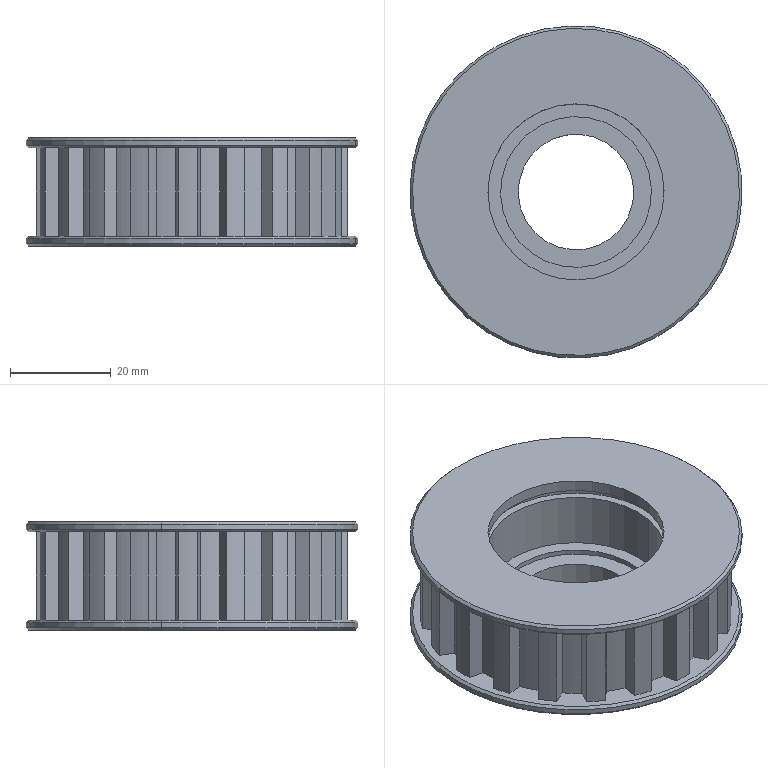Component | SolidWorks | DoubleFilmTransport-1_DrivenWheel-1 | 1 solid | 111 faces | volume 43508 mm3 | cylinder 55 | plane 48 | cone 8 | commonest cylinder face diameters 56 x21 62 x20 66 x4 35 x4 23 x2 30 x2 38 x2